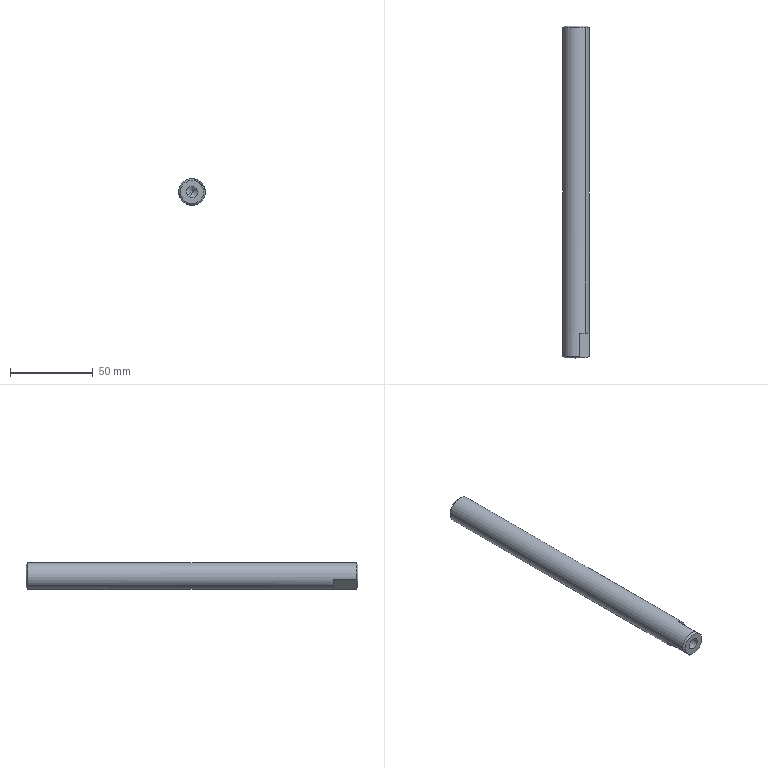Component | SolidWorks | PressingMechanism-14-1 | 1 solid | 16 faces | box 16 x 200 x 16 mm | volume 39181 mm3 | cone 6 | plane 6 | cylinder 4 | commonest cylinder face diameters 6.8 x2 16 x2
build123d program:
from build123d import *

# Parameters (mm, degrees)
SKETCH1_R             = 8
EXTRUDE1_DEPTH        = 200
M8_TAPPED_HOLE1_D     = 6.8
M8_TAPPED_HOLE1_DEPTH = 22.25
M8_TAPPED_HOLE1_TIP   = 2.043
CHAMFER1_SIZE         = 1
EXTRUDE2_DEPTH        = 201.32
EXTRUDE2_DEPTH_BACK   = 201.32
SKETCH4_W             = 15
SKETCH4_H             = 1


with BuildPart() as part:
    # Sketch1 → Extrude1 (new body)
    with BuildSketch(Plane(origin=(0, 0, 0), x_dir=(0, 0, -1), z_dir=(1, 0, 0))):
        Circle(SKETCH1_R)
    extrude(amount=EXTRUDE1_DEPTH)

    # M8 Tapped Hole1
    with Locations(Plane(origin=(200, 0, 0), x_dir=(0, 0, -1), z_dir=(1, 0, 0))):
        with Locations((0, 0)):
            Hole(M8_TAPPED_HOLE1_D / 2, depth=M8_TAPPED_HOLE1_DEPTH)
            with Locations((0, 0, -(M8_TAPPED_HOLE1_DEPTH + M8_TAPPED_HOLE1_TIP / 2))):  # 118° drill point
                Cone(0, M8_TAPPED_HOLE1_D / 2, M8_TAPPED_HOLE1_TIP, mode=Mode.SUBTRACT)

    # Chamfer1
    chamfer1_edges = [part.edges().sort_by_distance(p)[0] for p in [
        (0, 0, 8),
        (200, 0, 8),
    ]]
    chamfer(chamfer1_edges, length=CHAMFER1_SIZE)

    # Sketch4 → Extrude2 (cut, two sides: drawn at the far end of the back side and taken through both)
    with BuildSketch(Plane(origin=(0, 0, 0), x_dir=(1, 0, 0), z_dir=(0, 1, 0)).offset(-EXTRUDE2_DEPTH_BACK)):
        with Locations((192.5, 7.5)):
            Rectangle(SKETCH4_W, SKETCH4_H)
        with Locations((192.5, -7.5)):
            Rectangle(SKETCH4_W, SKETCH4_H)
    extrude(amount=EXTRUDE2_DEPTH + EXTRUDE2_DEPTH_BACK, mode=Mode.SUBTRACT)


solid = part.part

# Placed as in the assembly
solid = solid.moved(Location((191, -70.389, 100), (0, 45.184, -90)))
STEP:
#1=COLOUR_RGB('',0.7922,0.8196,0.9333);
#2=FILL_AREA_STYLE_COLOUR('',#1);
#3=FILL_AREA_STYLE('',(#2));
#4=SURFACE_STYLE_FILL_AREA(#3);
#5=SURFACE_SIDE_STYLE('',(#4));
#6=SURFACE_STYLE_USAGE(.BOTH.,#5);
#7=PRESENTATION_STYLE_ASSIGNMENT((#6));
#8=CARTESIAN_POINT('',(7.324,-2.771,3.743));
#9=VERTEX_POINT('',#8);
#10=CARTESIAN_POINT('',(7.715,-2.771,4.131));
#11=VERTEX_POINT('',#10);
#12=CARTESIAN_POINT('',(7.52,-2.771,3.937));
#13=DIRECTION('',(0.,1.,0.));
#14=DIRECTION('',(0.7094,0.,0.7048));
#15=AXIS2_PLACEMENT_3D('',#12,#13,#14);
#16=CIRCLE('',#15,0.2756);
#17=EDGE_CURVE('',#9,#11,#16,.T.);
#18=ORIENTED_EDGE('',*,*,#17,.F.);
#19=CARTESIAN_POINT('',(7.296,-2.811,3.715));
#20=VERTEX_POINT('',#19);
#21=CARTESIAN_POINT('',(7.296,-2.811,3.715));
#22=DIRECTION('',(-0.5016,-0.7071,-0.4984));
#23=VECTOR('',#22,39.37);
#24=LINE('',#21,#23);
#25=EDGE_CURVE('',#9,#20,#24,.T.);
#26=ORIENTED_EDGE('',*,*,#25,.T.);
#27=CARTESIAN_POINT('',(7.743,-2.811,4.159));
#28=VERTEX_POINT('',#27);
#29=CARTESIAN_POINT('',(7.52,-2.811,3.937));
#30=DIRECTION('',(0.,-1.,0.));
#31=DIRECTION('',(0.7094,0.,0.7048));
#32=AXIS2_PLACEMENT_3D('',#29,#30,#31);
#33=CIRCLE('',#32,0.315);
#34=EDGE_CURVE('',#28,#20,#33,.T.);
#35=ORIENTED_EDGE('',*,*,#34,.F.);
#36=CARTESIAN_POINT('',(7.743,-2.811,4.159));
#37=DIRECTION('',(0.5016,-0.7071,0.4984));
#38=VECTOR('',#37,39.37);
#39=LINE('',#36,#38);
#40=EDGE_CURVE('',#11,#28,#39,.T.);
#41=ORIENTED_EDGE('',*,*,#40,.F.);
#42=EDGE_LOOP('',(#18,#26,#35,#41));
#43=FACE_OUTER_BOUND('',#42,.T.);
#44=CARTESIAN_POINT('',(7.52,-2.811,3.937));
#45=DIRECTION('',(0.,-1.,0.));
#46=DIRECTION('',(0.7094,0.,0.7048));
#47=AXIS2_PLACEMENT_3D('',#44,#45,#46);
#48=CONICAL_SURFACE('',#47,0.315,0.7854);
#49=ADVANCED_FACE('',(#43),#48,.T.);
#50=CARTESIAN_POINT('',(7.425,-9.769,3.843));
#51=VERTEX_POINT('',#50);
#52=CARTESIAN_POINT('',(7.615,-9.769,4.031));
#53=VERTEX_POINT('',#52);
#54=CARTESIAN_POINT('',(7.52,-9.769,3.937));
#55=DIRECTION('',(0.,-1.,0.));
#56=DIRECTION('',(0.7094,0.,0.7048));
#57=AXIS2_PLACEMENT_3D('',#54,#55,#56);
#58=CIRCLE('',#57,0.1339);
#59=EDGE_CURVE('',#51,#53,#58,.T.);
#60=ORIENTED_EDGE('',*,*,#59,.F.);
#61=CARTESIAN_POINT('',(7.425,-10.645,3.843));
#62=VERTEX_POINT('',#61);
#63=CARTESIAN_POINT('',(7.425,-10.645,3.843));
#64=DIRECTION('',(0.,-1.,0.));
#65=VECTOR('',#64,39.37);
#66=LINE('',#63,#65);
#67=EDGE_CURVE('',#51,#62,#66,.T.);
#68=ORIENTED_EDGE('',*,*,#67,.T.);
#69=CARTESIAN_POINT('',(7.615,-10.645,4.031));
#70=VERTEX_POINT('',#69);
#71=CARTESIAN_POINT('',(7.52,-10.645,3.937));
#72=DIRECTION('',(0.,-1.,0.));
#73=DIRECTION('',(0.7094,0.,0.7048));
#74=AXIS2_PLACEMENT_3D('',#71,#72,#73);
#75=CIRCLE('',#74,0.1339);
#76=EDGE_CURVE('',#62,#70,#75,.T.);
#77=ORIENTED_EDGE('',*,*,#76,.T.);
#78=CARTESIAN_POINT('',(7.615,-10.645,4.031));
#79=DIRECTION('',(0.,-1.,0.));
#80=VECTOR('',#79,39.37);
#81=LINE('',#78,#80);
#82=EDGE_CURVE('',#53,#70,#81,.T.);
#83=ORIENTED_EDGE('',*,*,#82,.F.);
#84=EDGE_LOOP('',(#60,#68,#77,#83));
#85=FACE_OUTER_BOUND('',#84,.T.);
#86=CARTESIAN_POINT('',(7.52,-10.645,3.937));
#87=DIRECTION('',(0.,-1.,0.));
#88=DIRECTION('',(0.7094,0.,0.7048));
#89=AXIS2_PLACEMENT_3D('',#86,#87,#88);
#90=CYLINDRICAL_SURFACE('',#89,0.1339);
#91=ADVANCED_FACE('',(#85),#90,.F.);
#92=CARTESIAN_POINT('',(7.52,-9.689,3.937));
#93=VERTEX_POINT('',#92);
#94=CARTESIAN_POINT('',(7.615,-9.769,4.031));
#95=DIRECTION('',(0.608,-0.515,0.6042));
#96=VECTOR('',#95,39.37);
#97=LINE('',#94,#96);
#98=EDGE_CURVE('',#93,#53,#97,.T.);
#99=ORIENTED_EDGE('',*,*,#98,.F.);
#100=CARTESIAN_POINT('',(7.425,-9.769,3.843));
#101=DIRECTION('',(-0.608,-0.515,-0.6042));
#102=VECTOR('',#101,39.37);
#103=LINE('',#100,#102);
#104=EDGE_CURVE('',#93,#51,#103,.T.);
#105=ORIENTED_EDGE('',*,*,#104,.T.);
#106=ORIENTED_EDGE('',*,*,#59,.T.);
#107=EDGE_LOOP('',(#99,#105,#106));
#108=FACE_OUTER_BOUND('',#107,.T.);
#109=CARTESIAN_POINT('',(7.52,-9.769,3.937));
#110=DIRECTION('',(0.,-1.,0.));
#111=DIRECTION('',(0.7094,0.,0.7048));
#112=AXIS2_PLACEMENT_3D('',#109,#110,#111);
#113=CONICAL_SURFACE('',#112,0.1339,1.03);
#114=ADVANCED_FACE('',(#108),#113,.F.);
#115=CARTESIAN_POINT('',(7.608,-10.055,4.239));
#116=VERTEX_POINT('',#115);
#117=CARTESIAN_POINT('',(7.743,-10.055,4.159));
#118=VERTEX_POINT('',#117);
#119=CARTESIAN_POINT('',(7.52,-10.055,3.937));
#120=DIRECTION('',(0.,1.,0.));
#121=DIRECTION('',(-0.7094,0.,-0.7048));
#122=AXIS2_PLACEMENT_3D('',#119,#120,#121);
#123=CIRCLE('',#122,0.315);
#124=EDGE_CURVE('',#116,#118,#123,.T.);
#125=ORIENTED_EDGE('',*,*,#124,.T.);
#126=CARTESIAN_POINT('',(7.743,-10.645,4.159));
#127=DIRECTION('',(0.,1.,0.));
#128=VECTOR('',#127,39.37);
#129=LINE('',#126,#128);
#130=EDGE_CURVE('',#118,#28,#129,.T.);
#131=ORIENTED_EDGE('',*,*,#130,.T.);
#132=ORIENTED_EDGE('',*,*,#34,.T.);
#133=CARTESIAN_POINT('',(7.296,-10.055,3.715));
#134=VERTEX_POINT('',#133);
#135=CARTESIAN_POINT('',(7.296,-10.645,3.715));
#136=DIRECTION('',(0.,1.,0.));
#137=VECTOR('',#136,39.37);
#138=LINE('',#135,#137);
#139=EDGE_CURVE('',#134,#20,#138,.T.);
#140=ORIENTED_EDGE('',*,*,#139,.F.);
#141=CARTESIAN_POINT('',(7.217,-10.055,3.851));
#142=VERTEX_POINT('',#141);
#143=CARTESIAN_POINT('',(7.52,-10.055,3.937));
#144=DIRECTION('',(0.,1.,0.));
#145=DIRECTION('',(-0.7094,0.,-0.7048));
#146=AXIS2_PLACEMENT_3D('',#143,#144,#145);
#147=CIRCLE('',#146,0.315);
#148=EDGE_CURVE('',#134,#142,#147,.T.);
#149=ORIENTED_EDGE('',*,*,#148,.T.);
#150=CARTESIAN_POINT('',(7.217,-10.606,3.851));
#151=VERTEX_POINT('',#150);
#152=CARTESIAN_POINT('',(7.217,-10.645,3.851));
#153=DIRECTION('',(0.,-1.,0.));
#154=VECTOR('',#153,39.37);
#155=LINE('',#152,#154);
#156=EDGE_CURVE('',#142,#151,#155,.T.);
#157=ORIENTED_EDGE('',*,*,#156,.T.);
#158=CARTESIAN_POINT('',(7.608,-10.606,4.239));
#159=VERTEX_POINT('',#158);
#160=CARTESIAN_POINT('',(7.52,-10.606,3.937));
#161=DIRECTION('',(0.,1.,0.));
#162=DIRECTION('',(0.7094,0.,0.7048));
#163=AXIS2_PLACEMENT_3D('',#160,#161,#162);
#164=CIRCLE('',#163,0.315);
#165=EDGE_CURVE('',#151,#159,#164,.T.);
#166=ORIENTED_EDGE('',*,*,#165,.T.);
#167=CARTESIAN_POINT('',(7.608,-10.645,4.239));
#168=DIRECTION('',(0.,1.,0.));
#169=VECTOR('',#168,39.37);
#170=LINE('',#167,#169);
#171=EDGE_CURVE('',#159,#116,#170,.T.);
#172=ORIENTED_EDGE('',*,*,#171,.T.);
#173=EDGE_LOOP('',(#125,#131,#132,#140,#149,#157,#166,#172));
#174=FACE_OUTER_BOUND('',#173,.T.);
#175=CARTESIAN_POINT('',(7.52,-10.645,3.937));
#176=DIRECTION('',(0.,1.,0.));
#177=DIRECTION('',(-0.7094,0.,-0.7048));
#178=AXIS2_PLACEMENT_3D('',#175,#176,#177);
#179=CYLINDRICAL_SURFACE('',#178,0.315);
#180=ADVANCED_FACE('',(#174),#179,.T.);
#181=CARTESIAN_POINT('',(7.432,-10.606,3.635));
#182=VERTEX_POINT('',#181);
#183=CARTESIAN_POINT('',(7.324,-10.645,3.743));
#184=VERTEX_POINT('',#183);
#185=CARTESIAN_POINT('',(7.432,-10.606,3.635));
#186=CARTESIAN_POINT('',(7.415,-10.617,3.651));
#187=CARTESIAN_POINT('',(7.398,-10.627,3.669));
#188=CARTESIAN_POINT('',(7.362,-10.641,3.705));
#189=CARTESIAN_POINT('',(7.343,-10.645,3.724));
#190=CARTESIAN_POINT('',(7.324,-10.645,3.743));
#191=B_SPLINE_CURVE_WITH_KNOTS('',3,(#185,#186,#187,#188,#189,#190),.UNSPECIFIED.,.F.,.F.,(4,2,4),(0.02013,0.02213,0.02413),.UNSPECIFIED.);
#192=EDGE_CURVE('',#182,#184,#191,.T.);
#193=ORIENTED_EDGE('',*,*,#192,.F.);
#194=CARTESIAN_POINT('',(7.823,-10.606,4.023));
#195=VERTEX_POINT('',#194);
#196=CARTESIAN_POINT('',(7.52,-10.606,3.937));
#197=DIRECTION('',(0.,1.,0.));
#198=DIRECTION('',(0.7094,0.,0.7048));
#199=AXIS2_PLACEMENT_3D('',#196,#197,#198);
#200=CIRCLE('',#199,0.315);
#201=EDGE_CURVE('',#195,#182,#200,.T.);
#202=ORIENTED_EDGE('',*,*,#201,.F.);
#203=CARTESIAN_POINT('',(7.715,-10.645,4.131));
#204=VERTEX_POINT('',#203);
#205=CARTESIAN_POINT('',(7.715,-10.645,4.131));
#206=CARTESIAN_POINT('',(7.734,-10.645,4.112));
#207=CARTESIAN_POINT('',(7.753,-10.641,4.094));
#208=CARTESIAN_POINT('',(7.789,-10.627,4.057));
#209=CARTESIAN_POINT('',(7.806,-10.617,4.04));
#210=CARTESIAN_POINT('',(7.823,-10.606,4.023));
#211=B_SPLINE_CURVE_WITH_KNOTS('',3,(#205,#206,#207,#208,#209,#210),.UNSPECIFIED.,.F.,.F.,(4,2,4),(0.008364,0.01037,0.01237),.UNSPECIFIED.);
#212=EDGE_CURVE('',#204,#195,#211,.T.);
#213=ORIENTED_EDGE('',*,*,#212,.F.);
#214=CARTESIAN_POINT('',(7.52,-10.645,3.937));
#215=DIRECTION('',(0.,-1.,0.));
#216=DIRECTION('',(0.7094,0.,0.7048));
#217=AXIS2_PLACEMENT_3D('',#214,#215,#216);
#218=CIRCLE('',#217,0.2756);
#219=EDGE_CURVE('',#184,#204,#218,.T.);
#220=ORIENTED_EDGE('',*,*,#219,.F.);
#221=EDGE_LOOP('',(#193,#202,#213,#220));
#222=FACE_OUTER_BOUND('',#221,.T.);
#223=CARTESIAN_POINT('',(7.52,-10.645,3.937));
#224=DIRECTION('',(0.,1.,0.));
#225=DIRECTION('',(-0.7094,0.,-0.7048));
#226=AXIS2_PLACEMENT_3D('',#223,#224,#225);
#227=CONICAL_SURFACE('',#226,0.2756,0.7854);
#228=ADVANCED_FACE('',(#222),#227,.T.);
#229=ORIENTED_EDGE('',*,*,#130,.F.);
#230=CARTESIAN_POINT('',(7.823,-10.055,4.023));
#231=VERTEX_POINT('',#230);
#232=CARTESIAN_POINT('',(7.52,-10.055,3.937));
#233=DIRECTION('',(0.,1.,0.));
#234=DIRECTION('',(-0.7094,0.,-0.7048));
#235=AXIS2_PLACEMENT_3D('',#232,#233,#234);
#236=CIRCLE('',#235,0.315);
#237=EDGE_CURVE('',#118,#231,#236,.T.);
#238=ORIENTED_EDGE('',*,*,#237,.T.);
#239=CARTESIAN_POINT('',(7.823,-10.645,4.023));
#240=DIRECTION('',(0.,-1.,0.));
#241=VECTOR('',#240,39.37);
#242=LINE('',#239,#241);
#243=EDGE_CURVE('',#231,#195,#242,.T.);
#244=ORIENTED_EDGE('',*,*,#243,.T.);
#245=ORIENTED_EDGE('',*,*,#201,.T.);
#246=CARTESIAN_POINT('',(7.432,-10.055,3.635));
#247=VERTEX_POINT('',#246);
#248=CARTESIAN_POINT('',(7.432,-10.645,3.635));
#249=DIRECTION('',(0.,1.,0.));
#250=VECTOR('',#249,39.37);
#251=LINE('',#248,#250);
#252=EDGE_CURVE('',#182,#247,#251,.T.);
#253=ORIENTED_EDGE('',*,*,#252,.T.);
#254=CARTESIAN_POINT('',(7.52,-10.055,3.937));
#255=DIRECTION('',(0.,1.,0.));
#256=DIRECTION('',(-0.7094,0.,-0.7048));
#257=AXIS2_PLACEMENT_3D('',#254,#255,#256);
#258=CIRCLE('',#257,0.315);
#259=EDGE_CURVE('',#247,#134,#258,.T.);
#260=ORIENTED_EDGE('',*,*,#259,.T.);
#261=ORIENTED_EDGE('',*,*,#139,.T.);
#262=CARTESIAN_POINT('',(7.52,-2.811,3.937));
#263=DIRECTION('',(0.,-1.,0.));
#264=DIRECTION('',(0.7094,0.,0.7048));
#265=AXIS2_PLACEMENT_3D('',#262,#263,#264);
#266=CIRCLE('',#265,0.315);
#267=EDGE_CURVE('',#20,#28,#266,.T.);
#268=ORIENTED_EDGE('',*,*,#267,.T.);
#269=EDGE_LOOP('',(#229,#238,#244,#245,#253,#260,#261,#268));
#270=FACE_OUTER_BOUND('',#269,.T.);
#271=CARTESIAN_POINT('',(7.52,-10.645,3.937));
#272=DIRECTION('',(0.,1.,0.));
#273=DIRECTION('',(-0.7094,0.,-0.7048));
#274=AXIS2_PLACEMENT_3D('',#271,#272,#273);
#275=CYLINDRICAL_SURFACE('',#274,0.315);
#276=ADVANCED_FACE('',(#270),#275,.T.);
#277=CARTESIAN_POINT('',(7.52,-10.645,3.937));
#278=DIRECTION('',(0.,-1.,0.));
#279=DIRECTION('',(0.7094,0.,0.7048));
#280=AXIS2_PLACEMENT_3D('',#277,#278,#279);
#281=CIRCLE('',#280,0.2756);
#282=EDGE_CURVE('',#204,#184,#281,.T.);
#283=ORIENTED_EDGE('',*,*,#282,.T.);
#284=ORIENTED_EDGE('',*,*,#219,.T.);
#285=EDGE_LOOP('',(#283,#284));
#286=FACE_OUTER_BOUND('',#285,.T.);
#287=CARTESIAN_POINT('',(7.52,-10.645,3.937));
#288=DIRECTION('',(0.,-1.,0.));
#289=DIRECTION('',(0.7094,0.,0.7048));
#290=AXIS2_PLACEMENT_3D('',#287,#288,#289);
#291=CIRCLE('',#290,0.1339);
#292=EDGE_CURVE('',#70,#62,#291,.T.);
#293=ORIENTED_EDGE('',*,*,#292,.F.);
#294=ORIENTED_EDGE('',*,*,#76,.F.);
#295=EDGE_LOOP('',(#293,#294));
#296=FACE_BOUND('',#295,.T.);
#297=CARTESIAN_POINT('',(7.52,-10.645,3.937));
#298=DIRECTION('',(0.,-1.,0.));
#299=DIRECTION('',(0.7094,0.,0.7048));
#300=AXIS2_PLACEMENT_3D('',#297,#298,#299);
#301=PLANE('',#300);
#302=ADVANCED_FACE('',(#286,#296),#301,.T.);
#303=CARTESIAN_POINT('',(7.52,-2.771,3.937));
#304=DIRECTION('',(0.,1.,0.));
#305=DIRECTION('',(0.7094,0.,0.7048));
#306=AXIS2_PLACEMENT_3D('',#303,#304,#305);
#307=CIRCLE('',#306,0.2756);
#308=EDGE_CURVE('',#11,#9,#307,.T.);
#309=ORIENTED_EDGE('',*,*,#308,.T.);
#310=ORIENTED_EDGE('',*,*,#17,.T.);
#311=EDGE_LOOP('',(#309,#310));
#312=FACE_OUTER_BOUND('',#311,.T.);
#313=CARTESIAN_POINT('',(7.52,-2.771,3.937));
#314=DIRECTION('',(0.,-1.,0.));
#315=DIRECTION('',(0.7094,0.,0.7048));
#316=AXIS2_PLACEMENT_3D('',#313,#314,#315);
#317=PLANE('',#316);
#318=ADVANCED_FACE('',(#312),#317,.F.);
#319=ORIENTED_EDGE('',*,*,#104,.F.);
#320=ORIENTED_EDGE('',*,*,#98,.T.);
#321=CARTESIAN_POINT('',(7.52,-9.769,3.937));
#322=DIRECTION('',(0.,-1.,0.));
#323=DIRECTION('',(0.7094,0.,0.7048));
#324=AXIS2_PLACEMENT_3D('',#321,#322,#323);
#325=CIRCLE('',#324,0.1339);
#326=EDGE_CURVE('',#53,#51,#325,.T.);
#327=ORIENTED_EDGE('',*,*,#326,.T.);
#328=EDGE_LOOP('',(#319,#320,#327));
#329=FACE_OUTER_BOUND('',#328,.T.);
#330=CARTESIAN_POINT('',(7.52,-9.769,3.937));
#331=DIRECTION('',(0.,-1.,0.));
#332=DIRECTION('',(0.7094,0.,0.7048));
#333=AXIS2_PLACEMENT_3D('',#330,#331,#332);
#334=CONICAL_SURFACE('',#333,0.1339,1.03);
#335=ADVANCED_FACE('',(#329),#334,.F.);
#336=ORIENTED_EDGE('',*,*,#67,.F.);
#337=ORIENTED_EDGE('',*,*,#326,.F.);
#338=ORIENTED_EDGE('',*,*,#82,.T.);
#339=ORIENTED_EDGE('',*,*,#292,.T.);
#340=EDGE_LOOP('',(#336,#337,#338,#339));
#341=FACE_OUTER_BOUND('',#340,.T.);
#342=CARTESIAN_POINT('',(7.52,-10.645,3.937));
#343=DIRECTION('',(0.,-1.,0.));
#344=DIRECTION('',(0.7094,0.,0.7048));
#345=AXIS2_PLACEMENT_3D('',#342,#343,#344);
#346=CYLINDRICAL_SURFACE('',#345,0.1339);
#347=ADVANCED_FACE('',(#341),#346,.F.);
#348=ORIENTED_EDGE('',*,*,#25,.F.);
#349=ORIENTED_EDGE('',*,*,#308,.F.);
#350=ORIENTED_EDGE('',*,*,#40,.T.);
#351=ORIENTED_EDGE('',*,*,#267,.F.);
#352=EDGE_LOOP('',(#348,#349,#350,#351));
#353=FACE_OUTER_BOUND('',#352,.T.);
#354=CARTESIAN_POINT('',(7.52,-2.811,3.937));
#355=DIRECTION('',(0.,-1.,0.));
#356=DIRECTION('',(0.7094,0.,0.7048));
#357=AXIS2_PLACEMENT_3D('',#354,#355,#356);
#358=CONICAL_SURFACE('',#357,0.315,0.7854);
#359=ADVANCED_FACE('',(#353),#358,.T.);
#360=CARTESIAN_POINT('',(7.324,-10.645,3.743));
#361=CARTESIAN_POINT('',(7.315,-10.645,3.752));
#362=CARTESIAN_POINT('',(7.305,-10.644,3.762));
#363=CARTESIAN_POINT('',(7.287,-10.641,3.78));
#364=CARTESIAN_POINT('',(7.278,-10.638,3.789));
#365=CARTESIAN_POINT('',(7.26,-10.631,3.807));
#366=CARTESIAN_POINT('',(7.251,-10.627,3.816));
#367=CARTESIAN_POINT('',(7.234,-10.617,3.834));
#368=CARTESIAN_POINT('',(7.225,-10.612,3.843));
#369=CARTESIAN_POINT('',(7.217,-10.606,3.851));
#370=B_SPLINE_CURVE_WITH_KNOTS('',3,(#360,#361,#362,#363,#364,#365,#366,#367,#368,#369),.UNSPECIFIED.,.F.,.F.,(4,2,2,2,4),(0.02413,0.02513,0.02612,0.02712,0.02812),.UNSPECIFIED.);
#371=EDGE_CURVE('',#184,#151,#370,.T.);
#372=ORIENTED_EDGE('',*,*,#371,.F.);
#373=ORIENTED_EDGE('',*,*,#282,.F.);
#374=CARTESIAN_POINT('',(7.608,-10.606,4.239));
#375=CARTESIAN_POINT('',(7.616,-10.612,4.231));
#376=CARTESIAN_POINT('',(7.625,-10.617,4.222));
#377=CARTESIAN_POINT('',(7.642,-10.627,4.205));
#378=CARTESIAN_POINT('',(7.651,-10.631,4.196));
#379=CARTESIAN_POINT('',(7.669,-10.638,4.178));
#380=CARTESIAN_POINT('',(7.678,-10.641,4.169));
#381=CARTESIAN_POINT('',(7.696,-10.644,4.15));
#382=CARTESIAN_POINT('',(7.706,-10.645,4.141));
#383=CARTESIAN_POINT('',(7.715,-10.645,4.131));
#384=B_SPLINE_CURVE_WITH_KNOTS('',3,(#374,#375,#376,#377,#378,#379,#380,#381,#382,#383),.UNSPECIFIED.,.F.,.F.,(4,2,2,2,4),(0.004369,0.005367,0.006366,0.007365,0.008364),.UNSPECIFIED.);
#385=EDGE_CURVE('',#159,#204,#384,.T.);
#386=ORIENTED_EDGE('',*,*,#385,.F.);
#387=ORIENTED_EDGE('',*,*,#165,.F.);
#388=EDGE_LOOP('',(#372,#373,#386,#387));
#389=FACE_OUTER_BOUND('',#388,.T.);
#390=CARTESIAN_POINT('',(7.52,-10.645,3.937));
#391=DIRECTION('',(0.,1.,0.));
#392=DIRECTION('',(-0.7094,0.,-0.7048));
#393=AXIS2_PLACEMENT_3D('',#390,#391,#392);
#394=CONICAL_SURFACE('',#393,0.2756,0.7854);
#395=ADVANCED_FACE('',(#389),#394,.T.);
#396=CARTESIAN_POINT('',(7.937,-10.055,3.908));
#397=DIRECTION('',(-0.7048,0.,0.7094));
#398=VECTOR('',#397,39.37);
#399=LINE('',#396,#398);
#400=EDGE_CURVE('',#231,#116,#399,.T.);
#401=ORIENTED_EDGE('',*,*,#400,.F.);
#402=ORIENTED_EDGE('',*,*,#237,.F.);
#403=ORIENTED_EDGE('',*,*,#124,.F.);
#404=EDGE_LOOP('',(#401,#402,#403));
#405=FACE_OUTER_BOUND('',#404,.T.);
#406=CARTESIAN_POINT('',(7.937,-10.055,3.908));
#407=DIRECTION('',(0.,1.,0.));
#408=DIRECTION('',(-0.7094,0.,-0.7048));
#409=AXIS2_PLACEMENT_3D('',#406,#407,#408);
#410=PLANE('',#409);
#411=ADVANCED_FACE('',(#405),#410,.F.);
#412=ORIENTED_EDGE('',*,*,#385,.T.);
#413=ORIENTED_EDGE('',*,*,#212,.T.);
#414=ORIENTED_EDGE('',*,*,#243,.F.);
#415=ORIENTED_EDGE('',*,*,#400,.T.);
#416=ORIENTED_EDGE('',*,*,#171,.F.);
#417=EDGE_LOOP('',(#412,#413,#414,#415,#416));
#418=FACE_OUTER_BOUND('',#417,.T.);
#419=CARTESIAN_POINT('',(7.937,-10.645,3.908));
#420=DIRECTION('',(-0.7094,-0.,-0.7048));
#421=DIRECTION('',(0.,-1.,0.));
#422=AXIS2_PLACEMENT_3D('',#419,#420,#421);
#423=PLANE('',#422);
#424=ADVANCED_FACE('',(#418),#423,.F.);
#425=ORIENTED_EDGE('',*,*,#259,.F.);
#426=CARTESIAN_POINT('',(7.546,-10.055,3.519));
#427=DIRECTION('',(-0.7048,0.,0.7094));
#428=VECTOR('',#427,39.37);
#429=LINE('',#426,#428);
#430=EDGE_CURVE('',#247,#142,#429,.T.);
#431=ORIENTED_EDGE('',*,*,#430,.T.);
#432=ORIENTED_EDGE('',*,*,#148,.F.);
#433=EDGE_LOOP('',(#425,#431,#432));
#434=FACE_OUTER_BOUND('',#433,.T.);
#435=CARTESIAN_POINT('',(7.546,-10.055,3.519));
#436=DIRECTION('',(0.,1.,0.));
#437=DIRECTION('',(-0.7094,0.,-0.7048));
#438=AXIS2_PLACEMENT_3D('',#435,#436,#437);
#439=PLANE('',#438);
#440=ADVANCED_FACE('',(#434),#439,.F.);
#441=ORIENTED_EDGE('',*,*,#192,.T.);
#442=ORIENTED_EDGE('',*,*,#371,.T.);
#443=ORIENTED_EDGE('',*,*,#156,.F.);
#444=ORIENTED_EDGE('',*,*,#430,.F.);
#445=ORIENTED_EDGE('',*,*,#252,.F.);
#446=EDGE_LOOP('',(#441,#442,#443,#444,#445));
#447=FACE_OUTER_BOUND('',#446,.T.);
#448=CARTESIAN_POINT('',(7.546,-10.645,3.519));
#449=DIRECTION('',(0.7094,0.,0.7048));
#450=DIRECTION('',(-0.,1.,-0.));
#451=AXIS2_PLACEMENT_3D('',#448,#449,#450);
#452=PLANE('',#451);
#453=ADVANCED_FACE('',(#447),#452,.F.);
#454=CLOSED_SHELL('',(#49,#91,#114,#180,#228,#276,#302,#318,#335,#347,#359,#395,#411,#424,#440,#453));
#455=MANIFOLD_SOLID_BREP('',#454);
#456=STYLED_ITEM('',(#7),#455);
#457=(LENGTH_UNIT()NAMED_UNIT(*)SI_UNIT($,.METRE.));
#458=LENGTH_MEASURE_WITH_UNIT(LENGTH_MEASURE(0.0254),#457);
#459=DIMENSIONAL_EXPONENTS(1.,0.,0.,0.,0.,0.,0.);
#460=(CONVERSION_BASED_UNIT('',#458)LENGTH_UNIT()NAMED_UNIT(#459));
#461=UNCERTAINTY_MEASURE_WITH_UNIT(LENGTH_MEASURE(0.00001),#460,'','');
#462=(NAMED_UNIT(*)PLANE_ANGLE_UNIT()SI_UNIT($,.RADIAN.));
#463=(NAMED_UNIT(*)SI_UNIT($,.STERADIAN.)SOLID_ANGLE_UNIT());
#464=(GEOMETRIC_REPRESENTATION_CONTEXT(3)GLOBAL_UNCERTAINTY_ASSIGNED_CONTEXT((#461))GLOBAL_UNIT_ASSIGNED_CONTEXT((#460,#462,#463))REPRESENTATION_CONTEXT('',''));
#465=MECHANICAL_DESIGN_GEOMETRIC_PRESENTATION_REPRESENTATION('',(#456),#464);
#466=PRESENTATION_LAYER_ASSIGNMENT('','',(#456));
#467=CARTESIAN_POINT('',(0.,0.,0.));
#468=DIRECTION('',(0.,0.,1.));
#469=DIRECTION('',(1.,0.,0.));
#470=AXIS2_PLACEMENT_3D('',#467,#468,#469);
#471=(LENGTH_UNIT()NAMED_UNIT(*)SI_UNIT($,.METRE.));
#472=LENGTH_MEASURE_WITH_UNIT(LENGTH_MEASURE(0.0254),#471);
#473=DIMENSIONAL_EXPONENTS(1.,0.,0.,0.,0.,0.,0.);
#474=(CONVERSION_BASED_UNIT('',#472)LENGTH_UNIT()NAMED_UNIT(#473));
#475=UNCERTAINTY_MEASURE_WITH_UNIT(LENGTH_MEASURE(0.00001),#474,'','');
#476=(NAMED_UNIT(*)PLANE_ANGLE_UNIT()SI_UNIT($,.RADIAN.));
#477=(NAMED_UNIT(*)SI_UNIT($,.STERADIAN.)SOLID_ANGLE_UNIT());
#478=(GEOMETRIC_REPRESENTATION_CONTEXT(3)GLOBAL_UNCERTAINTY_ASSIGNED_CONTEXT((#475))GLOBAL_UNIT_ASSIGNED_CONTEXT((#474,#476,#477))REPRESENTATION_CONTEXT('',''));
#479=ADVANCED_BREP_SHAPE_REPRESENTATION('',(#455,#470),#478);